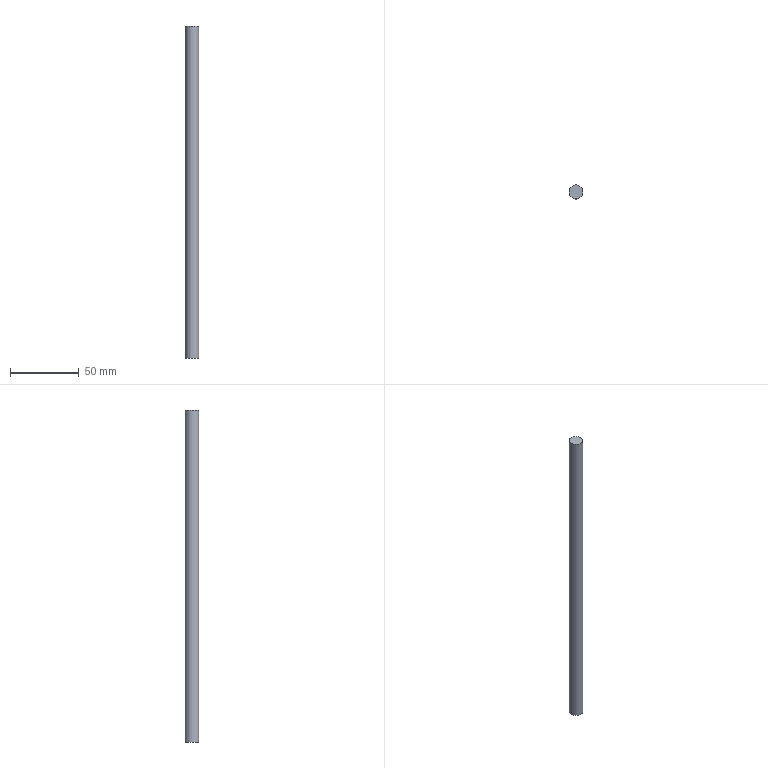Component | NX | STUD_2 | 1 solid | 3 faces | box 10 x 10 x 241 mm | volume 18928 mm3 | plane 2 | cylinder 1 | commonest cylinder face diameters 10 x1
STEP:
#1=CARTESIAN_POINT('',(0.,0.,0.));
#2=DIRECTION('',(0.,0.,1.));
#3=DIRECTION('',(1.,0.,0.));
#4=AXIS2_PLACEMENT_3D('',#1,#2,#3);
#5=CARTESIAN_POINT('',(-50.,-0.,177.5));
#6=VERTEX_POINT('',#5);
#7=CARTESIAN_POINT('',(-55.,-0.,177.5));
#8=DIRECTION('',(0.,0.,1.));
#9=DIRECTION('',(1.,0.,0.));
#10=AXIS2_PLACEMENT_3D('',#7,#8,#9);
#11=CIRCLE('',#10,5.);
#12=CARTESIAN_POINT('',(-55.,-0.,177.5));
#13=DIRECTION('',(0.,0.,-1.));
#14=DIRECTION('',(-1.,0.,0.));
#15=AXIS2_PLACEMENT_3D('',#12,#13,#14);
#16=CYLINDRICAL_SURFACE('',#15,5.);
#17=CARTESIAN_POINT('',(9.425,0.));
#18=DIRECTION('',(-1.,0.));
#19=VECTOR('',#18,1.);
#20=LINE('',#17,#19);
#21=(GEOMETRIC_REPRESENTATION_CONTEXT(2)PARAMETRIC_REPRESENTATION_CONTEXT()REPRESENTATION_CONTEXT('',''));
#22=DEFINITIONAL_REPRESENTATION('',(#20),#21);
#23=PCURVE('',#16,#22);
#24=CARTESIAN_POINT('',(-55.,-0.,177.5));
#25=DIRECTION('',(0.,0.,1.));
#26=DIRECTION('',(1.,0.,0.));
#27=AXIS2_PLACEMENT_3D('',#24,#25,#26);
#28=PLANE('',#27);
#29=CARTESIAN_POINT('',(0.,0.));
#30=DIRECTION('',(1.,0.));
#31=AXIS2_PLACEMENT_2D('',#29,#30);
#32=CIRCLE('',#31,5.);
#33=(GEOMETRIC_REPRESENTATION_CONTEXT(2)PARAMETRIC_REPRESENTATION_CONTEXT()REPRESENTATION_CONTEXT('',''));
#34=DEFINITIONAL_REPRESENTATION('',(#32),#33);
#35=PCURVE('',#28,#34);
#36=SURFACE_CURVE('',#11,(#23,#35),.PCURVE_S1.);
#37=EDGE_CURVE('',#6,#6,#36,.T.);
#38=ORIENTED_EDGE('',*,*,#37,.F.);
#39=CARTESIAN_POINT('',(-50.,-0.,-63.5));
#40=VERTEX_POINT('',#39);
#41=CARTESIAN_POINT('',(-50.,-0.,177.5));
#42=CARTESIAN_POINT('',(-50.,-0.,-63.5));
#43=B_SPLINE_CURVE_WITH_KNOTS('',1,(#41,#42),.UNSPECIFIED.,.F.,.F.,(2,2),(0.,241.),.PIECEWISE_BEZIER_KNOTS.);
#44=CARTESIAN_POINT('',(9.425,0.));
#45=DIRECTION('',(0.,1.));
#46=VECTOR('',#45,1.);
#47=LINE('',#44,#46);
#48=(GEOMETRIC_REPRESENTATION_CONTEXT(2)PARAMETRIC_REPRESENTATION_CONTEXT()REPRESENTATION_CONTEXT('',''));
#49=DEFINITIONAL_REPRESENTATION('',(#47),#48);
#50=PCURVE('',#16,#49);
#51=CARTESIAN_POINT('',(3.142,0.));
#52=DIRECTION('',(0.,1.));
#53=VECTOR('',#52,1.);
#54=LINE('',#51,#53);
#55=(GEOMETRIC_REPRESENTATION_CONTEXT(2)PARAMETRIC_REPRESENTATION_CONTEXT()REPRESENTATION_CONTEXT('',''));
#56=DEFINITIONAL_REPRESENTATION('',(#54),#55);
#57=PCURVE('',#16,#56);
#58=SEAM_CURVE('',#43,(#50,#57),.PCURVE_S1.);
#59=EDGE_CURVE('',#6,#40,#58,.T.);
#60=ORIENTED_EDGE('',*,*,#59,.T.);
#61=CARTESIAN_POINT('',(-55.,-0.,-63.5));
#62=DIRECTION('',(0.,0.,1.));
#63=DIRECTION('',(1.,0.,0.));
#64=AXIS2_PLACEMENT_3D('',#61,#62,#63);
#65=CIRCLE('',#64,5.);
#66=CARTESIAN_POINT('',(9.425,241.));
#67=DIRECTION('',(-1.,0.));
#68=VECTOR('',#67,1.);
#69=LINE('',#66,#68);
#70=(GEOMETRIC_REPRESENTATION_CONTEXT(2)PARAMETRIC_REPRESENTATION_CONTEXT()REPRESENTATION_CONTEXT('',''));
#71=DEFINITIONAL_REPRESENTATION('',(#69),#70);
#72=PCURVE('',#16,#71);
#73=CARTESIAN_POINT('',(-55.,-0.,-63.5));
#74=DIRECTION('',(0.,0.,1.));
#75=DIRECTION('',(1.,0.,0.));
#76=AXIS2_PLACEMENT_3D('',#73,#74,#75);
#77=PLANE('',#76);
#78=CARTESIAN_POINT('',(0.,0.));
#79=DIRECTION('',(1.,0.));
#80=AXIS2_PLACEMENT_2D('',#78,#79);
#81=CIRCLE('',#80,5.);
#82=(GEOMETRIC_REPRESENTATION_CONTEXT(2)PARAMETRIC_REPRESENTATION_CONTEXT()REPRESENTATION_CONTEXT('',''));
#83=DEFINITIONAL_REPRESENTATION('',(#81),#82);
#84=PCURVE('',#77,#83);
#85=SURFACE_CURVE('',#65,(#72,#84),.PCURVE_S1.);
#86=EDGE_CURVE('',#40,#40,#85,.T.);
#87=ORIENTED_EDGE('',*,*,#86,.T.);
#88=ORIENTED_EDGE('',*,*,#59,.F.);
#89=EDGE_LOOP('',(#38,#60,#87,#88));
#90=FACE_BOUND('',#89,.T.);
#91=ADVANCED_FACE('',(#90),#16,.T.);
#92=ORIENTED_EDGE('',*,*,#37,.T.);
#93=EDGE_LOOP('',(#92));
#94=FACE_BOUND('',#93,.T.);
#95=ADVANCED_FACE('',(#94),#28,.T.);
#96=ORIENTED_EDGE('',*,*,#86,.F.);
#97=EDGE_LOOP('',(#96));
#98=FACE_BOUND('',#97,.T.);
#99=ADVANCED_FACE('',(#98),#77,.F.);
#100=CLOSED_SHELL('',(#91,#95,#99));
#101=MANIFOLD_SOLID_BREP('',#100);
#102=(LENGTH_UNIT()NAMED_UNIT(*)SI_UNIT(.MILLI.,.METRE.));
#103=UNCERTAINTY_MEASURE_WITH_UNIT(LENGTH_MEASURE(0.00001),#102,'','');
#104=(NAMED_UNIT(*)PLANE_ANGLE_UNIT()SI_UNIT($,.RADIAN.));
#105=(NAMED_UNIT(*)SI_UNIT($,.STERADIAN.)SOLID_ANGLE_UNIT());
#106=(GEOMETRIC_REPRESENTATION_CONTEXT(3)GLOBAL_UNCERTAINTY_ASSIGNED_CONTEXT((#103))GLOBAL_UNIT_ASSIGNED_CONTEXT((#102,#104,#105))REPRESENTATION_CONTEXT('',''));
#107=ADVANCED_BREP_SHAPE_REPRESENTATION('',(#4,#101),#106);